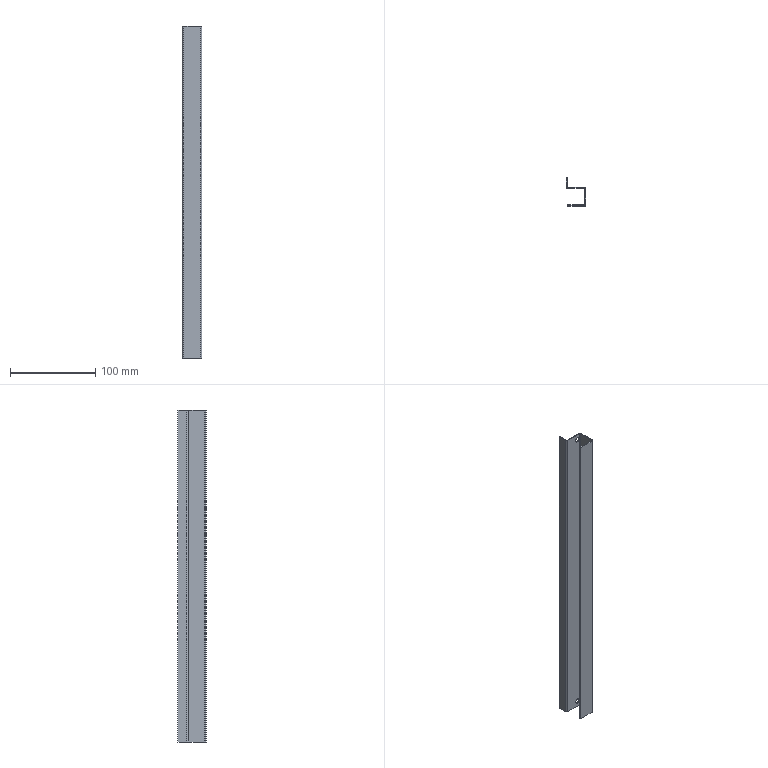Component | SolidWorks | CCQ-1.1-12LowerBeam2-2 | 1 solid | 34 faces | box 23 x 33 x 390 mm | volume 28572 mm3 | plane 24 | cylinder 10 | commonest cylinder face diameters 6 x4 1.473 x3 3.473 x3 | material 304
STEP:
#1=COLOUR_RGB('',0.7922,0.8196,0.9333);
#2=FILL_AREA_STYLE_COLOUR('',#1);
#3=FILL_AREA_STYLE('',(#2));
#4=SURFACE_STYLE_FILL_AREA(#3);
#5=SURFACE_SIDE_STYLE('',(#4));
#6=SURFACE_STYLE_USAGE(.BOTH.,#5);
#7=PRESENTATION_STYLE_ASSIGNMENT((#6));
#8=CARTESIAN_POINT('',(1.496,-17.185,-15.079));
#9=VERTEX_POINT('',#8);
#10=CARTESIAN_POINT('',(1.26,-17.185,-15.079));
#11=VERTEX_POINT('',#10);
#12=CARTESIAN_POINT('',(1.378,-17.185,-15.079));
#13=DIRECTION('',(0.,-1.,-0.));
#14=DIRECTION('',(-1.,0.,0.));
#15=AXIS2_PLACEMENT_3D('',#12,#13,#14);
#16=CIRCLE('',#15,0.1181);
#17=EDGE_CURVE('',#9,#11,#16,.T.);
#18=ORIENTED_EDGE('',*,*,#17,.T.);
#19=CARTESIAN_POINT('',(1.26,-17.146,-15.079));
#20=VERTEX_POINT('',#19);
#21=CARTESIAN_POINT('',(1.26,-17.539,-15.079));
#22=DIRECTION('',(-0.,1.,0.));
#23=VECTOR('',#22,39.37);
#24=LINE('',#21,#23);
#25=EDGE_CURVE('',#11,#20,#24,.T.);
#26=ORIENTED_EDGE('',*,*,#25,.T.);
#27=CARTESIAN_POINT('',(1.496,-17.146,-15.079));
#28=VERTEX_POINT('',#27);
#29=CARTESIAN_POINT('',(1.378,-17.146,-15.079));
#30=DIRECTION('',(-0.,1.,0.));
#31=DIRECTION('',(-1.,0.,0.));
#32=AXIS2_PLACEMENT_3D('',#29,#30,#31);
#33=CIRCLE('',#32,0.1181);
#34=EDGE_CURVE('',#20,#28,#33,.T.);
#35=ORIENTED_EDGE('',*,*,#34,.T.);
#36=CARTESIAN_POINT('',(1.496,-17.539,-15.079));
#37=DIRECTION('',(-0.,1.,0.));
#38=VECTOR('',#37,39.37);
#39=LINE('',#36,#38);
#40=EDGE_CURVE('',#9,#28,#39,.T.);
#41=ORIENTED_EDGE('',*,*,#40,.F.);
#42=EDGE_LOOP('',(#18,#26,#35,#41));
#43=FACE_OUTER_BOUND('',#42,.T.);
#44=CARTESIAN_POINT('',(1.378,-17.539,-15.079));
#45=DIRECTION('',(-0.,1.,0.));
#46=DIRECTION('',(1.,0.,0.));
#47=AXIS2_PLACEMENT_3D('',#44,#45,#46);
#48=CYLINDRICAL_SURFACE('',#47,0.1181);
#49=ADVANCED_FACE('',(#43),#48,.F.);
#50=CARTESIAN_POINT('',(1.496,-17.185,-0.2756));
#51=VERTEX_POINT('',#50);
#52=CARTESIAN_POINT('',(1.26,-17.185,-0.2756));
#53=VERTEX_POINT('',#52);
#54=CARTESIAN_POINT('',(1.378,-17.185,-0.2756));
#55=DIRECTION('',(0.,-1.,-0.));
#56=DIRECTION('',(-1.,0.,0.));
#57=AXIS2_PLACEMENT_3D('',#54,#55,#56);
#58=CIRCLE('',#57,0.1181);
#59=EDGE_CURVE('',#51,#53,#58,.T.);
#60=ORIENTED_EDGE('',*,*,#59,.T.);
#61=CARTESIAN_POINT('',(1.26,-17.146,-0.2756));
#62=VERTEX_POINT('',#61);
#63=CARTESIAN_POINT('',(1.26,-17.539,-0.2756));
#64=DIRECTION('',(-0.,1.,0.));
#65=VECTOR('',#64,39.37);
#66=LINE('',#63,#65);
#67=EDGE_CURVE('',#53,#62,#66,.T.);
#68=ORIENTED_EDGE('',*,*,#67,.T.);
#69=CARTESIAN_POINT('',(1.496,-17.146,-0.2756));
#70=VERTEX_POINT('',#69);
#71=CARTESIAN_POINT('',(1.378,-17.146,-0.2756));
#72=DIRECTION('',(-0.,1.,0.));
#73=DIRECTION('',(1.,0.,0.));
#74=AXIS2_PLACEMENT_3D('',#71,#72,#73);
#75=CIRCLE('',#74,0.1181);
#76=EDGE_CURVE('',#62,#70,#75,.T.);
#77=ORIENTED_EDGE('',*,*,#76,.T.);
#78=CARTESIAN_POINT('',(1.496,-17.539,-0.2756));
#79=DIRECTION('',(-0.,1.,0.));
#80=VECTOR('',#79,39.37);
#81=LINE('',#78,#80);
#82=EDGE_CURVE('',#51,#70,#81,.T.);
#83=ORIENTED_EDGE('',*,*,#82,.F.);
#84=EDGE_LOOP('',(#60,#68,#77,#83));
#85=FACE_OUTER_BOUND('',#84,.T.);
#86=CARTESIAN_POINT('',(1.378,-17.539,-0.2756));
#87=DIRECTION('',(-0.,1.,0.));
#88=DIRECTION('',(1.,0.,0.));
#89=AXIS2_PLACEMENT_3D('',#86,#87,#88);
#90=CYLINDRICAL_SURFACE('',#89,0.1181);
#91=ADVANCED_FACE('',(#85),#90,.F.);
#92=CARTESIAN_POINT('',(0.7377,-17.185,-15.354));
#93=VERTEX_POINT('',#92);
#94=CARTESIAN_POINT('',(0.7377,-17.146,-15.354));
#95=VERTEX_POINT('',#94);
#96=CARTESIAN_POINT('',(0.7377,-17.185,-15.354));
#97=DIRECTION('',(-0.,1.,0.));
#98=VECTOR('',#97,39.37);
#99=LINE('',#96,#98);
#100=EDGE_CURVE('',#93,#95,#99,.T.);
#101=ORIENTED_EDGE('',*,*,#100,.F.);
#102=CARTESIAN_POINT('',(0.6693,-17.117,-15.354));
#103=VERTEX_POINT('',#102);
#104=CARTESIAN_POINT('',(0.7377,-17.117,-15.354));
#105=DIRECTION('',(0.,0.,1.));
#106=DIRECTION('',(-1.,0.,0.));
#107=AXIS2_PLACEMENT_3D('',#104,#105,#106);
#108=CIRCLE('',#107,0.06837);
#109=EDGE_CURVE('',#103,#93,#108,.T.);
#110=ORIENTED_EDGE('',*,*,#109,.F.);
#111=CARTESIAN_POINT('',(0.7087,-17.117,-15.354));
#112=VERTEX_POINT('',#111);
#113=CARTESIAN_POINT('',(0.7087,-17.117,-15.354));
#114=DIRECTION('',(-1.,0.,-0.));
#115=VECTOR('',#114,39.37);
#116=LINE('',#113,#115);
#117=EDGE_CURVE('',#112,#103,#116,.T.);
#118=ORIENTED_EDGE('',*,*,#117,.F.);
#119=CARTESIAN_POINT('',(0.7377,-17.117,-15.354));
#120=DIRECTION('',(0.,0.,1.));
#121=DIRECTION('',(-1.,0.,0.));
#122=AXIS2_PLACEMENT_3D('',#119,#120,#121);
#123=CIRCLE('',#122,0.029);
#124=EDGE_CURVE('',#112,#95,#123,.T.);
#125=ORIENTED_EDGE('',*,*,#124,.T.);
#126=EDGE_LOOP('',(#101,#110,#118,#125));
#127=FACE_OUTER_BOUND('',#126,.T.);
#128=CARTESIAN_POINT('',(0.7377,-17.185,-15.354));
#129=DIRECTION('',(0.,-0.,-1.));
#130=DIRECTION('',(-1.,0.,-0.));
#131=AXIS2_PLACEMENT_3D('',#128,#129,#130);
#132=PLANE('',#131);
#133=ADVANCED_FACE('',(#127),#132,.T.);
#134=CARTESIAN_POINT('',(1.506,-17.185,-15.354));
#135=VERTEX_POINT('',#134);
#136=CARTESIAN_POINT('',(1.535,-17.185,-15.354));
#137=DIRECTION('',(1.,-0.,0.));
#138=VECTOR('',#137,39.37);
#139=LINE('',#136,#138);
#140=EDGE_CURVE('',#93,#135,#139,.T.);
#141=ORIENTED_EDGE('',*,*,#140,.F.);
#142=ORIENTED_EDGE('',*,*,#100,.T.);
#143=CARTESIAN_POINT('',(1.506,-17.146,-15.354));
#144=VERTEX_POINT('',#143);
#145=CARTESIAN_POINT('',(1.535,-17.146,-15.354));
#146=DIRECTION('',(1.,-0.,0.));
#147=VECTOR('',#146,39.37);
#148=LINE('',#145,#147);
#149=EDGE_CURVE('',#95,#144,#148,.T.);
#150=ORIENTED_EDGE('',*,*,#149,.T.);
#151=CARTESIAN_POINT('',(1.506,-17.146,-15.354));
#152=DIRECTION('',(0.,-1.,-0.));
#153=VECTOR('',#152,39.37);
#154=LINE('',#151,#153);
#155=EDGE_CURVE('',#144,#135,#154,.T.);
#156=ORIENTED_EDGE('',*,*,#155,.T.);
#157=EDGE_LOOP('',(#141,#142,#150,#156));
#158=FACE_OUTER_BOUND('',#157,.T.);
#159=CARTESIAN_POINT('',(0.7087,-17.117,-15.354));
#160=DIRECTION('',(0.,-0.,-1.));
#161=DIRECTION('',(-1.,0.,-0.));
#162=AXIS2_PLACEMENT_3D('',#159,#160,#161);
#163=PLANE('',#162);
#164=ADVANCED_FACE('',(#158),#163,.T.);
#165=CARTESIAN_POINT('',(0.6693,-17.117,0.));
#166=VERTEX_POINT('',#165);
#167=CARTESIAN_POINT('',(0.7087,-17.117,0.));
#168=VERTEX_POINT('',#167);
#169=CARTESIAN_POINT('',(0.6693,-17.117,0.));
#170=DIRECTION('',(1.,-0.,0.));
#171=VECTOR('',#170,39.37);
#172=LINE('',#169,#171);
#173=EDGE_CURVE('',#166,#168,#172,.T.);
#174=ORIENTED_EDGE('',*,*,#173,.F.);
#175=CARTESIAN_POINT('',(0.7377,-17.185,0.));
#176=VERTEX_POINT('',#175);
#177=CARTESIAN_POINT('',(0.7377,-17.117,0.));
#178=DIRECTION('',(0.,0.,1.));
#179=DIRECTION('',(-1.,0.,-0.));
#180=AXIS2_PLACEMENT_3D('',#177,#178,#179);
#181=CIRCLE('',#180,0.06837);
#182=EDGE_CURVE('',#166,#176,#181,.T.);
#183=ORIENTED_EDGE('',*,*,#182,.T.);
#184=CARTESIAN_POINT('',(0.7377,-17.146,0.));
#185=VERTEX_POINT('',#184);
#186=CARTESIAN_POINT('',(0.7377,-17.146,0.));
#187=DIRECTION('',(0.,-1.,-0.));
#188=VECTOR('',#187,39.37);
#189=LINE('',#186,#188);
#190=EDGE_CURVE('',#185,#176,#189,.T.);
#191=ORIENTED_EDGE('',*,*,#190,.F.);
#192=CARTESIAN_POINT('',(0.7377,-17.117,0.));
#193=DIRECTION('',(0.,0.,1.));
#194=DIRECTION('',(-1.,0.,-0.));
#195=AXIS2_PLACEMENT_3D('',#192,#193,#194);
#196=CIRCLE('',#195,0.029);
#197=EDGE_CURVE('',#168,#185,#196,.T.);
#198=ORIENTED_EDGE('',*,*,#197,.F.);
#199=EDGE_LOOP('',(#174,#183,#191,#198));
#200=FACE_OUTER_BOUND('',#199,.T.);
#201=CARTESIAN_POINT('',(0.6693,-17.117,0.));
#202=DIRECTION('',(-0.,0.,1.));
#203=DIRECTION('',(1.,-0.,0.));
#204=AXIS2_PLACEMENT_3D('',#201,#202,#203);
#205=PLANE('',#204);
#206=ADVANCED_FACE('',(#200),#205,.T.);
#207=CARTESIAN_POINT('',(0.6693,-16.713,0.));
#208=VERTEX_POINT('',#207);
#209=CARTESIAN_POINT('',(0.6693,-17.185,0.));
#210=DIRECTION('',(0.,-1.,-0.));
#211=VECTOR('',#210,39.37);
#212=LINE('',#209,#211);
#213=EDGE_CURVE('',#208,#166,#212,.T.);
#214=ORIENTED_EDGE('',*,*,#213,.T.);
#215=ORIENTED_EDGE('',*,*,#173,.T.);
#216=CARTESIAN_POINT('',(0.7087,-16.713,0.));
#217=VERTEX_POINT('',#216);
#218=CARTESIAN_POINT('',(0.7087,-17.185,0.));
#219=DIRECTION('',(0.,-1.,-0.));
#220=VECTOR('',#219,39.37);
#221=LINE('',#218,#220);
#222=EDGE_CURVE('',#217,#168,#221,.T.);
#223=ORIENTED_EDGE('',*,*,#222,.F.);
#224=CARTESIAN_POINT('',(0.7087,-16.713,0.));
#225=DIRECTION('',(-1.,0.,-0.));
#226=VECTOR('',#225,39.37);
#227=LINE('',#224,#226);
#228=EDGE_CURVE('',#217,#208,#227,.T.);
#229=ORIENTED_EDGE('',*,*,#228,.T.);
#230=EDGE_LOOP('',(#214,#215,#223,#229));
#231=FACE_OUTER_BOUND('',#230,.T.);
#232=CARTESIAN_POINT('',(0.7377,-17.146,0.));
#233=DIRECTION('',(-0.,0.,1.));
#234=DIRECTION('',(1.,-0.,0.));
#235=AXIS2_PLACEMENT_3D('',#232,#233,#234);
#236=PLANE('',#235);
#237=ADVANCED_FACE('',(#231),#236,.T.);
#238=CARTESIAN_POINT('',(1.535,-17.214,-15.354));
#239=VERTEX_POINT('',#238);
#240=CARTESIAN_POINT('',(1.575,-17.214,-15.354));
#241=VERTEX_POINT('',#240);
#242=CARTESIAN_POINT('',(1.535,-17.214,-15.354));
#243=DIRECTION('',(1.,-0.,0.));
#244=VECTOR('',#243,39.37);
#245=LINE('',#242,#244);
#246=EDGE_CURVE('',#239,#241,#245,.T.);
#247=ORIENTED_EDGE('',*,*,#246,.F.);
#248=CARTESIAN_POINT('',(1.506,-17.214,-15.354));
#249=DIRECTION('',(-0.,-0.,-1.));
#250=DIRECTION('',(1.,0.,0.));
#251=AXIS2_PLACEMENT_3D('',#248,#249,#250);
#252=CIRCLE('',#251,0.029);
#253=EDGE_CURVE('',#135,#239,#252,.T.);
#254=ORIENTED_EDGE('',*,*,#253,.F.);
#255=ORIENTED_EDGE('',*,*,#155,.F.);
#256=CARTESIAN_POINT('',(1.506,-17.214,-15.354));
#257=DIRECTION('',(-0.,-0.,-1.));
#258=DIRECTION('',(-1.,0.,0.));
#259=AXIS2_PLACEMENT_3D('',#256,#257,#258);
#260=CIRCLE('',#259,0.06837);
#261=EDGE_CURVE('',#144,#241,#260,.T.);
#262=ORIENTED_EDGE('',*,*,#261,.T.);
#263=EDGE_LOOP('',(#247,#254,#255,#262));
#264=FACE_OUTER_BOUND('',#263,.T.);
#265=CARTESIAN_POINT('',(1.535,-17.214,-15.354));
#266=DIRECTION('',(0.,-0.,-1.));
#267=DIRECTION('',(-1.,0.,-0.));
#268=AXIS2_PLACEMENT_3D('',#265,#266,#267);
#269=PLANE('',#268);
#270=ADVANCED_FACE('',(#264),#269,.T.);
#271=CARTESIAN_POINT('',(1.535,-17.943,-15.354));
#272=VERTEX_POINT('',#271);
#273=CARTESIAN_POINT('',(1.535,-17.972,-15.354));
#274=DIRECTION('',(0.,-1.,-0.));
#275=VECTOR('',#274,39.37);
#276=LINE('',#273,#275);
#277=EDGE_CURVE('',#239,#272,#276,.T.);
#278=ORIENTED_EDGE('',*,*,#277,.F.);
#279=ORIENTED_EDGE('',*,*,#246,.T.);
#280=CARTESIAN_POINT('',(1.575,-17.943,-15.354));
#281=VERTEX_POINT('',#280);
#282=CARTESIAN_POINT('',(1.575,-17.972,-15.354));
#283=DIRECTION('',(0.,-1.,-0.));
#284=VECTOR('',#283,39.37);
#285=LINE('',#282,#284);
#286=EDGE_CURVE('',#241,#281,#285,.T.);
#287=ORIENTED_EDGE('',*,*,#286,.T.);
#288=CARTESIAN_POINT('',(1.575,-17.943,-15.354));
#289=DIRECTION('',(-1.,0.,-0.));
#290=VECTOR('',#289,39.37);
#291=LINE('',#288,#290);
#292=EDGE_CURVE('',#281,#272,#291,.T.);
#293=ORIENTED_EDGE('',*,*,#292,.T.);
#294=EDGE_LOOP('',(#278,#279,#287,#293));
#295=FACE_OUTER_BOUND('',#294,.T.);
#296=CARTESIAN_POINT('',(1.506,-17.146,-15.354));
#297=DIRECTION('',(0.,-0.,-1.));
#298=DIRECTION('',(-1.,0.,-0.));
#299=AXIS2_PLACEMENT_3D('',#296,#297,#298);
#300=PLANE('',#299);
#301=ADVANCED_FACE('',(#295),#300,.T.);
#302=CARTESIAN_POINT('',(1.506,-17.185,0.));
#303=VERTEX_POINT('',#302);
#304=CARTESIAN_POINT('',(1.506,-17.146,0.));
#305=VERTEX_POINT('',#304);
#306=CARTESIAN_POINT('',(1.506,-17.185,0.));
#307=DIRECTION('',(-0.,1.,0.));
#308=VECTOR('',#307,39.37);
#309=LINE('',#306,#308);
#310=EDGE_CURVE('',#303,#305,#309,.T.);
#311=ORIENTED_EDGE('',*,*,#310,.F.);
#312=CARTESIAN_POINT('',(1.535,-17.214,0.));
#313=VERTEX_POINT('',#312);
#314=CARTESIAN_POINT('',(1.506,-17.214,0.));
#315=DIRECTION('',(-0.,-0.,-1.));
#316=DIRECTION('',(1.,0.,0.));
#317=AXIS2_PLACEMENT_3D('',#314,#315,#316);
#318=CIRCLE('',#317,0.029);
#319=EDGE_CURVE('',#303,#313,#318,.T.);
#320=ORIENTED_EDGE('',*,*,#319,.T.);
#321=CARTESIAN_POINT('',(1.575,-17.214,0.));
#322=VERTEX_POINT('',#321);
#323=CARTESIAN_POINT('',(1.575,-17.214,0.));
#324=DIRECTION('',(-1.,0.,-0.));
#325=VECTOR('',#324,39.37);
#326=LINE('',#323,#325);
#327=EDGE_CURVE('',#322,#313,#326,.T.);
#328=ORIENTED_EDGE('',*,*,#327,.F.);
#329=CARTESIAN_POINT('',(1.506,-17.214,0.));
#330=DIRECTION('',(-0.,-0.,-1.));
#331=DIRECTION('',(-1.,0.,-0.));
#332=AXIS2_PLACEMENT_3D('',#329,#330,#331);
#333=CIRCLE('',#332,0.06837);
#334=EDGE_CURVE('',#305,#322,#333,.T.);
#335=ORIENTED_EDGE('',*,*,#334,.F.);
#336=EDGE_LOOP('',(#311,#320,#328,#335));
#337=FACE_OUTER_BOUND('',#336,.T.);
#338=CARTESIAN_POINT('',(1.506,-17.185,0.));
#339=DIRECTION('',(-0.,0.,1.));
#340=DIRECTION('',(1.,-0.,0.));
#341=AXIS2_PLACEMENT_3D('',#338,#339,#340);
#342=PLANE('',#341);
#343=ADVANCED_FACE('',(#337),#342,.T.);
#344=CARTESIAN_POINT('',(1.535,-17.185,0.));
#345=DIRECTION('',(1.,-0.,0.));
#346=VECTOR('',#345,39.37);
#347=LINE('',#344,#346);
#348=EDGE_CURVE('',#176,#303,#347,.T.);
#349=ORIENTED_EDGE('',*,*,#348,.T.);
#350=ORIENTED_EDGE('',*,*,#310,.T.);
#351=CARTESIAN_POINT('',(1.535,-17.146,0.));
#352=DIRECTION('',(1.,-0.,0.));
#353=VECTOR('',#352,39.37);
#354=LINE('',#351,#353);
#355=EDGE_CURVE('',#185,#305,#354,.T.);
#356=ORIENTED_EDGE('',*,*,#355,.F.);
#357=ORIENTED_EDGE('',*,*,#190,.T.);
#358=EDGE_LOOP('',(#349,#350,#356,#357));
#359=FACE_OUTER_BOUND('',#358,.T.);
#360=CARTESIAN_POINT('',(1.575,-17.214,0.));
#361=DIRECTION('',(-0.,0.,1.));
#362=DIRECTION('',(1.,-0.,0.));
#363=AXIS2_PLACEMENT_3D('',#360,#361,#362);
#364=PLANE('',#363);
#365=ADVANCED_FACE('',(#359),#364,.T.);
#366=CARTESIAN_POINT('',(1.506,-17.972,-15.354));
#367=VERTEX_POINT('',#366);
#368=CARTESIAN_POINT('',(1.506,-18.012,-15.354));
#369=VERTEX_POINT('',#368);
#370=CARTESIAN_POINT('',(1.506,-17.972,-15.354));
#371=DIRECTION('',(0.,-1.,-0.));
#372=VECTOR('',#371,39.37);
#373=LINE('',#370,#372);
#374=EDGE_CURVE('',#367,#369,#373,.T.);
#375=ORIENTED_EDGE('',*,*,#374,.F.);
#376=CARTESIAN_POINT('',(1.506,-17.943,-15.354));
#377=DIRECTION('',(-0.,-0.,-1.));
#378=DIRECTION('',(1.,0.,0.));
#379=AXIS2_PLACEMENT_3D('',#376,#377,#378);
#380=CIRCLE('',#379,0.029);
#381=EDGE_CURVE('',#272,#367,#380,.T.);
#382=ORIENTED_EDGE('',*,*,#381,.F.);
#383=ORIENTED_EDGE('',*,*,#292,.F.);
#384=CARTESIAN_POINT('',(1.506,-17.943,-15.354));
#385=DIRECTION('',(-0.,-0.,-1.));
#386=DIRECTION('',(-1.,0.,0.));
#387=AXIS2_PLACEMENT_3D('',#384,#385,#386);
#388=CIRCLE('',#387,0.06837);
#389=EDGE_CURVE('',#281,#369,#388,.T.);
#390=ORIENTED_EDGE('',*,*,#389,.T.);
#391=EDGE_LOOP('',(#375,#382,#383,#390));
#392=FACE_OUTER_BOUND('',#391,.T.);
#393=CARTESIAN_POINT('',(1.506,-17.972,-15.354));
#394=DIRECTION('',(0.,-0.,-1.));
#395=DIRECTION('',(-1.,0.,-0.));
#396=AXIS2_PLACEMENT_3D('',#393,#394,#395);
#397=PLANE('',#396);
#398=ADVANCED_FACE('',(#392),#397,.T.);
#399=CARTESIAN_POINT('',(0.748,-17.972,-15.354));
#400=VERTEX_POINT('',#399);
#401=CARTESIAN_POINT('',(1.535,-17.972,-15.354));
#402=DIRECTION('',(-1.,0.,-0.));
#403=VECTOR('',#402,39.37);
#404=LINE('',#401,#403);
#405=EDGE_CURVE('',#367,#400,#404,.T.);
#406=ORIENTED_EDGE('',*,*,#405,.F.);
#407=ORIENTED_EDGE('',*,*,#374,.T.);
#408=CARTESIAN_POINT('',(0.748,-18.012,-15.354));
#409=VERTEX_POINT('',#408);
#410=CARTESIAN_POINT('',(1.535,-18.012,-15.354));
#411=DIRECTION('',(-1.,0.,-0.));
#412=VECTOR('',#411,39.37);
#413=LINE('',#410,#412);
#414=EDGE_CURVE('',#369,#409,#413,.T.);
#415=ORIENTED_EDGE('',*,*,#414,.T.);
#416=CARTESIAN_POINT('',(0.748,-17.972,-15.354));
#417=DIRECTION('',(0.,-1.,-0.));
#418=VECTOR('',#417,39.37);
#419=LINE('',#416,#418);
#420=EDGE_CURVE('',#400,#409,#419,.T.);
#421=ORIENTED_EDGE('',*,*,#420,.F.);
#422=EDGE_LOOP('',(#406,#407,#415,#421));
#423=FACE_OUTER_BOUND('',#422,.T.);
#424=CARTESIAN_POINT('',(1.575,-17.943,-15.354));
#425=DIRECTION('',(0.,-0.,-1.));
#426=DIRECTION('',(-1.,0.,-0.));
#427=AXIS2_PLACEMENT_3D('',#424,#425,#426);
#428=PLANE('',#427);
#429=ADVANCED_FACE('',(#423),#428,.T.);
#430=CARTESIAN_POINT('',(1.535,-17.943,0.));
#431=VERTEX_POINT('',#430);
#432=CARTESIAN_POINT('',(1.575,-17.943,0.));
#433=VERTEX_POINT('',#432);
#434=CARTESIAN_POINT('',(1.535,-17.943,0.));
#435=DIRECTION('',(1.,-0.,0.));
#436=VECTOR('',#435,39.37);
#437=LINE('',#434,#436);
#438=EDGE_CURVE('',#431,#433,#437,.T.);
#439=ORIENTED_EDGE('',*,*,#438,.F.);
#440=CARTESIAN_POINT('',(1.506,-17.972,0.));
#441=VERTEX_POINT('',#440);
#442=CARTESIAN_POINT('',(1.506,-17.943,0.));
#443=DIRECTION('',(-0.,-0.,-1.));
#444=DIRECTION('',(1.,0.,0.));
#445=AXIS2_PLACEMENT_3D('',#442,#443,#444);
#446=CIRCLE('',#445,0.029);
#447=EDGE_CURVE('',#431,#441,#446,.T.);
#448=ORIENTED_EDGE('',*,*,#447,.T.);
#449=CARTESIAN_POINT('',(1.506,-18.012,0.));
#450=VERTEX_POINT('',#449);
#451=CARTESIAN_POINT('',(1.506,-18.012,0.));
#452=DIRECTION('',(-0.,1.,0.));
#453=VECTOR('',#452,39.37);
#454=LINE('',#451,#453);
#455=EDGE_CURVE('',#450,#441,#454,.T.);
#456=ORIENTED_EDGE('',*,*,#455,.F.);
#457=CARTESIAN_POINT('',(1.506,-17.943,0.));
#458=DIRECTION('',(-0.,-0.,-1.));
#459=DIRECTION('',(-1.,0.,-0.));
#460=AXIS2_PLACEMENT_3D('',#457,#458,#459);
#461=CIRCLE('',#460,0.06837);
#462=EDGE_CURVE('',#433,#450,#461,.T.);
#463=ORIENTED_EDGE('',*,*,#462,.F.);
#464=EDGE_LOOP('',(#439,#448,#456,#463));
#465=FACE_OUTER_BOUND('',#464,.T.);
#466=CARTESIAN_POINT('',(1.535,-17.943,0.));
#467=DIRECTION('',(-0.,0.,1.));
#468=DIRECTION('',(1.,-0.,0.));
#469=AXIS2_PLACEMENT_3D('',#466,#467,#468);
#470=PLANE('',#469);
#471=ADVANCED_FACE('',(#465),#470,.T.);
#472=CARTESIAN_POINT('',(1.535,-17.972,0.));
#473=DIRECTION('',(0.,-1.,-0.));
#474=VECTOR('',#473,39.37);
#475=LINE('',#472,#474);
#476=EDGE_CURVE('',#313,#431,#475,.T.);
#477=ORIENTED_EDGE('',*,*,#476,.T.);
#478=ORIENTED_EDGE('',*,*,#438,.T.);
#479=CARTESIAN_POINT('',(1.575,-17.972,0.));
#480=DIRECTION('',(0.,-1.,-0.));
#481=VECTOR('',#480,39.37);
#482=LINE('',#479,#481);
#483=EDGE_CURVE('',#322,#433,#482,.T.);
#484=ORIENTED_EDGE('',*,*,#483,.F.);
#485=ORIENTED_EDGE('',*,*,#327,.T.);
#486=EDGE_LOOP('',(#477,#478,#484,#485));
#487=FACE_OUTER_BOUND('',#486,.T.);
#488=CARTESIAN_POINT('',(1.506,-18.012,0.));
#489=DIRECTION('',(-0.,0.,1.));
#490=DIRECTION('',(1.,-0.,0.));
#491=AXIS2_PLACEMENT_3D('',#488,#489,#490);
#492=PLANE('',#491);
#493=ADVANCED_FACE('',(#487),#492,.T.);
#494=CARTESIAN_POINT('',(0.748,-18.012,0.));
#495=VERTEX_POINT('',#494);
#496=CARTESIAN_POINT('',(1.535,-18.012,0.));
#497=DIRECTION('',(-1.,0.,-0.));
#498=VECTOR('',#497,39.37);
#499=LINE('',#496,#498);
#500=EDGE_CURVE('',#450,#495,#499,.T.);
#501=ORIENTED_EDGE('',*,*,#500,.T.);
#502=CARTESIAN_POINT('',(0.748,-18.012,-15.354));
#503=DIRECTION('',(0.,0.,1.));
#504=VECTOR('',#503,39.37);
#505=LINE('',#502,#504);
#506=EDGE_CURVE('',#409,#495,#505,.T.);
#507=ORIENTED_EDGE('',*,*,#506,.F.);
#508=ORIENTED_EDGE('',*,*,#414,.F.);
#509=CARTESIAN_POINT('',(1.506,-18.012,-15.354));
#510=DIRECTION('',(0.,0.,1.));
#511=VECTOR('',#510,39.37);
#512=LINE('',#509,#511);
#513=EDGE_CURVE('',#369,#450,#512,.T.);
#514=ORIENTED_EDGE('',*,*,#513,.T.);
#515=EDGE_LOOP('',(#501,#507,#508,#514));
#516=FACE_OUTER_BOUND('',#515,.T.);
#517=CARTESIAN_POINT('',(1.535,-18.012,-15.354));
#518=DIRECTION('',(0.,1.,0.));
#519=DIRECTION('',(1.,-0.,0.));
#520=AXIS2_PLACEMENT_3D('',#517,#518,#519);
#521=PLANE('',#520);
#522=ADVANCED_FACE('',(#516),#521,.F.);
#523=CARTESIAN_POINT('',(0.748,-17.972,0.));
#524=VERTEX_POINT('',#523);
#525=CARTESIAN_POINT('',(0.748,-17.972,0.));
#526=DIRECTION('',(0.,-1.,-0.));
#527=VECTOR('',#526,39.37);
#528=LINE('',#525,#527);
#529=EDGE_CURVE('',#524,#495,#528,.T.);
#530=ORIENTED_EDGE('',*,*,#529,.F.);
#531=CARTESIAN_POINT('',(0.748,-17.972,-15.354));
#532=DIRECTION('',(0.,0.,1.));
#533=VECTOR('',#532,39.37);
#534=LINE('',#531,#533);
#535=EDGE_CURVE('',#400,#524,#534,.T.);
#536=ORIENTED_EDGE('',*,*,#535,.F.);
#537=ORIENTED_EDGE('',*,*,#420,.T.);
#538=ORIENTED_EDGE('',*,*,#506,.T.);
#539=EDGE_LOOP('',(#530,#536,#537,#538));
#540=FACE_OUTER_BOUND('',#539,.T.);
#541=CARTESIAN_POINT('',(0.748,-17.972,-15.354));
#542=DIRECTION('',(-1.,0.,0.));
#543=DIRECTION('',(0.,0.,1.));
#544=AXIS2_PLACEMENT_3D('',#541,#542,#543);
#545=PLANE('',#544);
#546=ADVANCED_FACE('',(#540),#545,.T.);
#547=CARTESIAN_POINT('',(1.535,-17.972,0.));
#548=DIRECTION('',(-1.,0.,-0.));
#549=VECTOR('',#548,39.37);
#550=LINE('',#547,#549);
#551=EDGE_CURVE('',#441,#524,#550,.T.);
#552=ORIENTED_EDGE('',*,*,#551,.F.);
#553=CARTESIAN_POINT('',(1.506,-17.972,-15.354));
#554=DIRECTION('',(0.,0.,1.));
#555=VECTOR('',#554,39.37);
#556=LINE('',#553,#555);
#557=EDGE_CURVE('',#367,#441,#556,.T.);
#558=ORIENTED_EDGE('',*,*,#557,.F.);
#559=ORIENTED_EDGE('',*,*,#405,.T.);
#560=ORIENTED_EDGE('',*,*,#535,.T.);
#561=EDGE_LOOP('',(#552,#558,#559,#560));
#562=FACE_OUTER_BOUND('',#561,.T.);
#563=CARTESIAN_POINT('',(1.535,-17.972,-15.354));
#564=DIRECTION('',(0.,1.,0.));
#565=DIRECTION('',(1.,-0.,0.));
#566=AXIS2_PLACEMENT_3D('',#563,#564,#565);
#567=PLANE('',#566);
#568=ADVANCED_FACE('',(#562),#567,.T.);
#569=ORIENTED_EDGE('',*,*,#447,.F.);
#570=CARTESIAN_POINT('',(1.535,-17.943,-15.354));
#571=DIRECTION('',(0.,0.,1.));
#572=VECTOR('',#571,39.37);
#573=LINE('',#570,#572);
#574=EDGE_CURVE('',#272,#431,#573,.T.);
#575=ORIENTED_EDGE('',*,*,#574,.F.);
#576=ORIENTED_EDGE('',*,*,#381,.T.);
#577=ORIENTED_EDGE('',*,*,#557,.T.);
#578=EDGE_LOOP('',(#569,#575,#576,#577));
#579=FACE_OUTER_BOUND('',#578,.T.);
#580=CARTESIAN_POINT('',(1.506,-17.943,-15.354));
#581=DIRECTION('',(0.,0.,1.));
#582=DIRECTION('',(1.,0.,0.));
#583=AXIS2_PLACEMENT_3D('',#580,#581,#582);
#584=CYLINDRICAL_SURFACE('',#583,0.029);
#585=ADVANCED_FACE('',(#579),#584,.F.);
#586=ORIENTED_EDGE('',*,*,#476,.F.);
#587=CARTESIAN_POINT('',(1.535,-17.214,-15.354));
#588=DIRECTION('',(0.,0.,1.));
#589=VECTOR('',#588,39.37);
#590=LINE('',#587,#589);
#591=EDGE_CURVE('',#239,#313,#590,.T.);
#592=ORIENTED_EDGE('',*,*,#591,.F.);
#593=ORIENTED_EDGE('',*,*,#277,.T.);
#594=ORIENTED_EDGE('',*,*,#574,.T.);
#595=EDGE_LOOP('',(#586,#592,#593,#594));
#596=FACE_OUTER_BOUND('',#595,.T.);
#597=CARTESIAN_POINT('',(1.535,-17.972,-15.354));
#598=DIRECTION('',(-1.,0.,0.));
#599=DIRECTION('',(0.,0.,1.));
#600=AXIS2_PLACEMENT_3D('',#597,#598,#599);
#601=PLANE('',#600);
#602=ADVANCED_FACE('',(#596),#601,.T.);
#603=ORIENTED_EDGE('',*,*,#319,.F.);
#604=CARTESIAN_POINT('',(1.506,-17.185,-15.354));
#605=DIRECTION('',(0.,0.,1.));
#606=VECTOR('',#605,39.37);
#607=LINE('',#604,#606);
#608=EDGE_CURVE('',#135,#303,#607,.T.);
#609=ORIENTED_EDGE('',*,*,#608,.F.);
#610=ORIENTED_EDGE('',*,*,#253,.T.);
#611=ORIENTED_EDGE('',*,*,#591,.T.);
#612=EDGE_LOOP('',(#603,#609,#610,#611));
#613=FACE_OUTER_BOUND('',#612,.T.);
#614=CARTESIAN_POINT('',(1.506,-17.214,-15.354));
#615=DIRECTION('',(0.,0.,1.));
#616=DIRECTION('',(1.,0.,0.));
#617=AXIS2_PLACEMENT_3D('',#614,#615,#616);
#618=CYLINDRICAL_SURFACE('',#617,0.029);
#619=ADVANCED_FACE('',(#613),#618,.F.);
#620=ORIENTED_EDGE('',*,*,#17,.F.);
#621=CARTESIAN_POINT('',(1.378,-17.185,-15.079));
#622=DIRECTION('',(0.,-1.,-0.));
#623=DIRECTION('',(-1.,0.,0.));
#624=AXIS2_PLACEMENT_3D('',#621,#622,#623);
#625=CIRCLE('',#624,0.1181);
#626=EDGE_CURVE('',#11,#9,#625,.T.);
#627=ORIENTED_EDGE('',*,*,#626,.F.);
#628=EDGE_LOOP('',(#620,#627));
#629=FACE_BOUND('',#628,.T.);
#630=ORIENTED_EDGE('',*,*,#59,.F.);
#631=CARTESIAN_POINT('',(1.378,-17.185,-0.2756));
#632=DIRECTION('',(0.,-1.,-0.));
#633=DIRECTION('',(-1.,0.,0.));
#634=AXIS2_PLACEMENT_3D('',#631,#632,#633);
#635=CIRCLE('',#634,0.1181);
#636=EDGE_CURVE('',#53,#51,#635,.T.);
#637=ORIENTED_EDGE('',*,*,#636,.F.);
#638=EDGE_LOOP('',(#630,#637));
#639=FACE_BOUND('',#638,.T.);
#640=ORIENTED_EDGE('',*,*,#348,.F.);
#641=CARTESIAN_POINT('',(0.7377,-17.185,-15.354));
#642=DIRECTION('',(0.,0.,1.));
#643=VECTOR('',#642,39.37);
#644=LINE('',#641,#643);
#645=EDGE_CURVE('',#93,#176,#644,.T.);
#646=ORIENTED_EDGE('',*,*,#645,.F.);
#647=ORIENTED_EDGE('',*,*,#140,.T.);
#648=ORIENTED_EDGE('',*,*,#608,.T.);
#649=EDGE_LOOP('',(#640,#646,#647,#648));
#650=FACE_OUTER_BOUND('',#649,.T.);
#651=CARTESIAN_POINT('',(1.535,-17.185,-15.354));
#652=DIRECTION('',(-0.,-1.,-0.));
#653=DIRECTION('',(-1.,0.,-0.));
#654=AXIS2_PLACEMENT_3D('',#651,#652,#653);
#655=PLANE('',#654);
#656=ADVANCED_FACE('',(#629,#639,#650),#655,.T.);
#657=ORIENTED_EDGE('',*,*,#182,.F.);
#658=CARTESIAN_POINT('',(0.6693,-17.117,-15.354));
#659=DIRECTION('',(0.,0.,1.));
#660=VECTOR('',#659,39.37);
#661=LINE('',#658,#660);
#662=EDGE_CURVE('',#103,#166,#661,.T.);
#663=ORIENTED_EDGE('',*,*,#662,.F.);
#664=ORIENTED_EDGE('',*,*,#109,.T.);
#665=ORIENTED_EDGE('',*,*,#645,.T.);
#666=EDGE_LOOP('',(#657,#663,#664,#665));
#667=FACE_OUTER_BOUND('',#666,.T.);
#668=CARTESIAN_POINT('',(0.7377,-17.117,-15.354));
#669=DIRECTION('',(0.,0.,1.));
#670=DIRECTION('',(1.,0.,0.));
#671=AXIS2_PLACEMENT_3D('',#668,#669,#670);
#672=CYLINDRICAL_SURFACE('',#671,0.06837);
#673=ADVANCED_FACE('',(#667),#672,.T.);
#674=ORIENTED_EDGE('',*,*,#213,.F.);
#675=CARTESIAN_POINT('',(0.6693,-16.713,-15.354));
#676=VERTEX_POINT('',#675);
#677=CARTESIAN_POINT('',(0.6693,-16.713,-15.354));
#678=DIRECTION('',(0.,0.,1.));
#679=VECTOR('',#678,39.37);
#680=LINE('',#677,#679);
#681=EDGE_CURVE('',#676,#208,#680,.T.);
#682=ORIENTED_EDGE('',*,*,#681,.F.);
#683=CARTESIAN_POINT('',(0.6693,-17.185,-15.354));
#684=DIRECTION('',(0.,-1.,-0.));
#685=VECTOR('',#684,39.37);
#686=LINE('',#683,#685);
#687=EDGE_CURVE('',#676,#103,#686,.T.);
#688=ORIENTED_EDGE('',*,*,#687,.T.);
#689=ORIENTED_EDGE('',*,*,#662,.T.);
#690=EDGE_LOOP('',(#674,#682,#688,#689));
#691=FACE_OUTER_BOUND('',#690,.T.);
#692=CARTESIAN_POINT('',(0.6693,-17.185,-15.354));
#693=DIRECTION('',(-1.,0.,0.));
#694=DIRECTION('',(0.,0.,1.));
#695=AXIS2_PLACEMENT_3D('',#692,#693,#694);
#696=PLANE('',#695);
#697=ADVANCED_FACE('',(#691),#696,.T.);
#698=ORIENTED_EDGE('',*,*,#228,.F.);
#699=CARTESIAN_POINT('',(0.7087,-16.713,-15.354));
#700=VERTEX_POINT('',#699);
#701=CARTESIAN_POINT('',(0.7087,-16.713,-15.354));
#702=DIRECTION('',(0.,0.,1.));
#703=VECTOR('',#702,39.37);
#704=LINE('',#701,#703);
#705=EDGE_CURVE('',#700,#217,#704,.T.);
#706=ORIENTED_EDGE('',*,*,#705,.F.);
#707=CARTESIAN_POINT('',(0.7087,-16.713,-15.354));
#708=DIRECTION('',(-1.,0.,-0.));
#709=VECTOR('',#708,39.37);
#710=LINE('',#707,#709);
#711=EDGE_CURVE('',#700,#676,#710,.T.);
#712=ORIENTED_EDGE('',*,*,#711,.T.);
#713=ORIENTED_EDGE('',*,*,#681,.T.);
#714=EDGE_LOOP('',(#698,#706,#712,#713));
#715=FACE_OUTER_BOUND('',#714,.T.);
#716=CARTESIAN_POINT('',(0.7087,-16.713,-15.354));
#717=DIRECTION('',(0.,1.,0.));
#718=DIRECTION('',(1.,-0.,0.));
#719=AXIS2_PLACEMENT_3D('',#716,#717,#718);
#720=PLANE('',#719);
#721=ADVANCED_FACE('',(#715),#720,.T.);
#722=ORIENTED_EDGE('',*,*,#222,.T.);
#723=CARTESIAN_POINT('',(0.7087,-17.117,-15.354));
#724=DIRECTION('',(0.,0.,1.));
#725=VECTOR('',#724,39.37);
#726=LINE('',#723,#725);
#727=EDGE_CURVE('',#112,#168,#726,.T.);
#728=ORIENTED_EDGE('',*,*,#727,.F.);
#729=CARTESIAN_POINT('',(0.7087,-17.185,-15.354));
#730=DIRECTION('',(0.,-1.,-0.));
#731=VECTOR('',#730,39.37);
#732=LINE('',#729,#731);
#733=EDGE_CURVE('',#700,#112,#732,.T.);
#734=ORIENTED_EDGE('',*,*,#733,.F.);
#735=ORIENTED_EDGE('',*,*,#705,.T.);
#736=EDGE_LOOP('',(#722,#728,#734,#735));
#737=FACE_OUTER_BOUND('',#736,.T.);
#738=CARTESIAN_POINT('',(0.7087,-17.185,-15.354));
#739=DIRECTION('',(-1.,0.,0.));
#740=DIRECTION('',(0.,0.,1.));
#741=AXIS2_PLACEMENT_3D('',#738,#739,#740);
#742=PLANE('',#741);
#743=ADVANCED_FACE('',(#737),#742,.F.);
#744=ORIENTED_EDGE('',*,*,#197,.T.);
#745=CARTESIAN_POINT('',(0.7377,-17.146,-15.354));
#746=DIRECTION('',(0.,0.,1.));
#747=VECTOR('',#746,39.37);
#748=LINE('',#745,#747);
#749=EDGE_CURVE('',#95,#185,#748,.T.);
#750=ORIENTED_EDGE('',*,*,#749,.F.);
#751=ORIENTED_EDGE('',*,*,#124,.F.);
#752=ORIENTED_EDGE('',*,*,#727,.T.);
#753=EDGE_LOOP('',(#744,#750,#751,#752));
#754=FACE_OUTER_BOUND('',#753,.T.);
#755=CARTESIAN_POINT('',(0.7377,-17.117,-15.354));
#756=DIRECTION('',(0.,0.,1.));
#757=DIRECTION('',(1.,0.,0.));
#758=AXIS2_PLACEMENT_3D('',#755,#756,#757);
#759=CYLINDRICAL_SURFACE('',#758,0.029);
#760=ADVANCED_FACE('',(#754),#759,.F.);
#761=CARTESIAN_POINT('',(1.378,-17.146,-15.079));
#762=DIRECTION('',(-0.,1.,0.));
#763=DIRECTION('',(-1.,0.,0.));
#764=AXIS2_PLACEMENT_3D('',#761,#762,#763);
#765=CIRCLE('',#764,0.1181);
#766=EDGE_CURVE('',#28,#20,#765,.T.);
#767=ORIENTED_EDGE('',*,*,#766,.F.);
#768=ORIENTED_EDGE('',*,*,#34,.F.);
#769=EDGE_LOOP('',(#767,#768));
#770=FACE_BOUND('',#769,.T.);
#771=CARTESIAN_POINT('',(1.378,-17.146,-0.2756));
#772=DIRECTION('',(-0.,1.,0.));
#773=DIRECTION('',(1.,0.,0.));
#774=AXIS2_PLACEMENT_3D('',#771,#772,#773);
#775=CIRCLE('',#774,0.1181);
#776=EDGE_CURVE('',#70,#62,#775,.T.);
#777=ORIENTED_EDGE('',*,*,#776,.F.);
#778=ORIENTED_EDGE('',*,*,#76,.F.);
#779=EDGE_LOOP('',(#777,#778));
#780=FACE_BOUND('',#779,.T.);
#781=ORIENTED_EDGE('',*,*,#355,.T.);
#782=CARTESIAN_POINT('',(1.506,-17.146,-15.354));
#783=DIRECTION('',(0.,0.,1.));
#784=VECTOR('',#783,39.37);
#785=LINE('',#782,#784);
#786=EDGE_CURVE('',#144,#305,#785,.T.);
#787=ORIENTED_EDGE('',*,*,#786,.F.);
#788=ORIENTED_EDGE('',*,*,#149,.F.);
#789=ORIENTED_EDGE('',*,*,#749,.T.);
#790=EDGE_LOOP('',(#781,#787,#788,#789));
#791=FACE_OUTER_BOUND('',#790,.T.);
#792=CARTESIAN_POINT('',(1.535,-17.146,-15.354));
#793=DIRECTION('',(-0.,-1.,-0.));
#794=DIRECTION('',(-1.,0.,-0.));
#795=AXIS2_PLACEMENT_3D('',#792,#793,#794);
#796=PLANE('',#795);
#797=ADVANCED_FACE('',(#770,#780,#791),#796,.F.);
#798=ORIENTED_EDGE('',*,*,#334,.T.);
#799=CARTESIAN_POINT('',(1.575,-17.214,-15.354));
#800=DIRECTION('',(0.,0.,1.));
#801=VECTOR('',#800,39.37);
#802=LINE('',#799,#801);
#803=EDGE_CURVE('',#241,#322,#802,.T.);
#804=ORIENTED_EDGE('',*,*,#803,.F.);
#805=ORIENTED_EDGE('',*,*,#261,.F.);
#806=ORIENTED_EDGE('',*,*,#786,.T.);
#807=EDGE_LOOP('',(#798,#804,#805,#806));
#808=FACE_OUTER_BOUND('',#807,.T.);
#809=CARTESIAN_POINT('',(1.506,-17.214,-15.354));
#810=DIRECTION('',(0.,0.,1.));
#811=DIRECTION('',(1.,0.,0.));
#812=AXIS2_PLACEMENT_3D('',#809,#810,#811);
#813=CYLINDRICAL_SURFACE('',#812,0.06837);
#814=ADVANCED_FACE('',(#808),#813,.T.);
#815=ORIENTED_EDGE('',*,*,#483,.T.);
#816=CARTESIAN_POINT('',(1.575,-17.943,-15.354));
#817=DIRECTION('',(0.,0.,1.));
#818=VECTOR('',#817,39.37);
#819=LINE('',#816,#818);
#820=EDGE_CURVE('',#281,#433,#819,.T.);
#821=ORIENTED_EDGE('',*,*,#820,.F.);
#822=ORIENTED_EDGE('',*,*,#286,.F.);
#823=ORIENTED_EDGE('',*,*,#803,.T.);
#824=EDGE_LOOP('',(#815,#821,#822,#823));
#825=FACE_OUTER_BOUND('',#824,.T.);
#826=CARTESIAN_POINT('',(1.575,-17.972,-15.354));
#827=DIRECTION('',(-1.,0.,0.));
#828=DIRECTION('',(0.,0.,1.));
#829=AXIS2_PLACEMENT_3D('',#826,#827,#828);
#830=PLANE('',#829);
#831=ADVANCED_FACE('',(#825),#830,.F.);
#832=ORIENTED_EDGE('',*,*,#462,.T.);
#833=ORIENTED_EDGE('',*,*,#513,.F.);
#834=ORIENTED_EDGE('',*,*,#389,.F.);
#835=ORIENTED_EDGE('',*,*,#820,.T.);
#836=EDGE_LOOP('',(#832,#833,#834,#835));
#837=FACE_OUTER_BOUND('',#836,.T.);
#838=CARTESIAN_POINT('',(1.506,-17.943,-15.354));
#839=DIRECTION('',(0.,0.,1.));
#840=DIRECTION('',(1.,0.,0.));
#841=AXIS2_PLACEMENT_3D('',#838,#839,#840);
#842=CYLINDRICAL_SURFACE('',#841,0.06837);
#843=ADVANCED_FACE('',(#837),#842,.T.);
#844=ORIENTED_EDGE('',*,*,#733,.T.);
#845=ORIENTED_EDGE('',*,*,#117,.T.);
#846=ORIENTED_EDGE('',*,*,#687,.F.);
#847=ORIENTED_EDGE('',*,*,#711,.F.);
#848=EDGE_LOOP('',(#844,#845,#846,#847));
#849=FACE_OUTER_BOUND('',#848,.T.);
#850=CARTESIAN_POINT('',(1.506,-17.943,-15.354));
#851=DIRECTION('',(-0.,0.,1.));
#852=DIRECTION('',(1.,-0.,0.));
#853=AXIS2_PLACEMENT_3D('',#850,#851,#852);
#854=PLANE('',#853);
#855=ADVANCED_FACE('',(#849),#854,.F.);
#856=ORIENTED_EDGE('',*,*,#500,.F.);
#857=ORIENTED_EDGE('',*,*,#455,.T.);
#858=ORIENTED_EDGE('',*,*,#551,.T.);
#859=ORIENTED_EDGE('',*,*,#529,.T.);
#860=EDGE_LOOP('',(#856,#857,#858,#859));
#861=FACE_OUTER_BOUND('',#860,.T.);
#862=CARTESIAN_POINT('',(1.506,-17.943,0.));
#863=DIRECTION('',(-0.,0.,1.));
#864=DIRECTION('',(1.,-0.,0.));
#865=AXIS2_PLACEMENT_3D('',#862,#863,#864);
#866=PLANE('',#865);
#867=ADVANCED_FACE('',(#861),#866,.T.);
#868=ORIENTED_EDGE('',*,*,#67,.F.);
#869=ORIENTED_EDGE('',*,*,#636,.T.);
#870=ORIENTED_EDGE('',*,*,#82,.T.);
#871=ORIENTED_EDGE('',*,*,#776,.T.);
#872=EDGE_LOOP('',(#868,#869,#870,#871));
#873=FACE_OUTER_BOUND('',#872,.T.);
#874=CARTESIAN_POINT('',(1.378,-17.539,-0.2756));
#875=DIRECTION('',(-0.,1.,0.));
#876=DIRECTION('',(1.,0.,0.));
#877=AXIS2_PLACEMENT_3D('',#874,#875,#876);
#878=CYLINDRICAL_SURFACE('',#877,0.1181);
#879=ADVANCED_FACE('',(#873),#878,.F.);
#880=ORIENTED_EDGE('',*,*,#25,.F.);
#881=ORIENTED_EDGE('',*,*,#626,.T.);
#882=ORIENTED_EDGE('',*,*,#40,.T.);
#883=ORIENTED_EDGE('',*,*,#766,.T.);
#884=EDGE_LOOP('',(#880,#881,#882,#883));
#885=FACE_OUTER_BOUND('',#884,.T.);
#886=CARTESIAN_POINT('',(1.378,-17.539,-15.079));
#887=DIRECTION('',(-0.,1.,0.));
#888=DIRECTION('',(1.,0.,0.));
#889=AXIS2_PLACEMENT_3D('',#886,#887,#888);
#890=CYLINDRICAL_SURFACE('',#889,0.1181);
#891=ADVANCED_FACE('',(#885),#890,.F.);
#892=CLOSED_SHELL('',(#49,#91,#133,#164,#206,#237,#270,#301,#343,#365,#398,#429,#471,#493,#522,#546,#568,#585,#602,#619,#656,#673,#697,#721,#743,#760,#797,#814,#831,#843,#855,#867,#879,#891));
#893=MANIFOLD_SOLID_BREP('',#892);
#894=STYLED_ITEM('',(#7),#893);
#895=(LENGTH_UNIT()NAMED_UNIT(*)SI_UNIT($,.METRE.));
#896=LENGTH_MEASURE_WITH_UNIT(LENGTH_MEASURE(0.0254),#895);
#897=DIMENSIONAL_EXPONENTS(1.,0.,0.,0.,0.,0.,0.);
#898=(CONVERSION_BASED_UNIT('',#896)LENGTH_UNIT()NAMED_UNIT(#897));
#899=UNCERTAINTY_MEASURE_WITH_UNIT(LENGTH_MEASURE(0.00001),#898,'','');
#900=(NAMED_UNIT(*)PLANE_ANGLE_UNIT()SI_UNIT($,.RADIAN.));
#901=(NAMED_UNIT(*)SI_UNIT($,.STERADIAN.)SOLID_ANGLE_UNIT());
#902=(GEOMETRIC_REPRESENTATION_CONTEXT(3)GLOBAL_UNCERTAINTY_ASSIGNED_CONTEXT((#899))GLOBAL_UNIT_ASSIGNED_CONTEXT((#898,#900,#901))REPRESENTATION_CONTEXT('',''));
#903=MECHANICAL_DESIGN_GEOMETRIC_PRESENTATION_REPRESENTATION('',(#894),#902);
#904=CARTESIAN_POINT('',(0.,0.,0.));
#905=DIRECTION('',(0.,0.,1.));
#906=DIRECTION('',(1.,0.,0.));
#907=AXIS2_PLACEMENT_3D('',#904,#905,#906);
#908=(LENGTH_UNIT()NAMED_UNIT(*)SI_UNIT($,.METRE.));
#909=LENGTH_MEASURE_WITH_UNIT(LENGTH_MEASURE(0.0254),#908);
#910=DIMENSIONAL_EXPONENTS(1.,0.,0.,0.,0.,0.,0.);
#911=(CONVERSION_BASED_UNIT('',#909)LENGTH_UNIT()NAMED_UNIT(#910));
#912=UNCERTAINTY_MEASURE_WITH_UNIT(LENGTH_MEASURE(0.00001),#911,'','');
#913=(NAMED_UNIT(*)PLANE_ANGLE_UNIT()SI_UNIT($,.RADIAN.));
#914=(NAMED_UNIT(*)SI_UNIT($,.STERADIAN.)SOLID_ANGLE_UNIT());
#915=(GEOMETRIC_REPRESENTATION_CONTEXT(3)GLOBAL_UNCERTAINTY_ASSIGNED_CONTEXT((#912))GLOBAL_UNIT_ASSIGNED_CONTEXT((#911,#913,#914))REPRESENTATION_CONTEXT('',''));
#916=ADVANCED_BREP_SHAPE_REPRESENTATION('',(#893,#907),#915);
#917=PRESENTATION_LAYER_ASSIGNMENT('','',(#894));